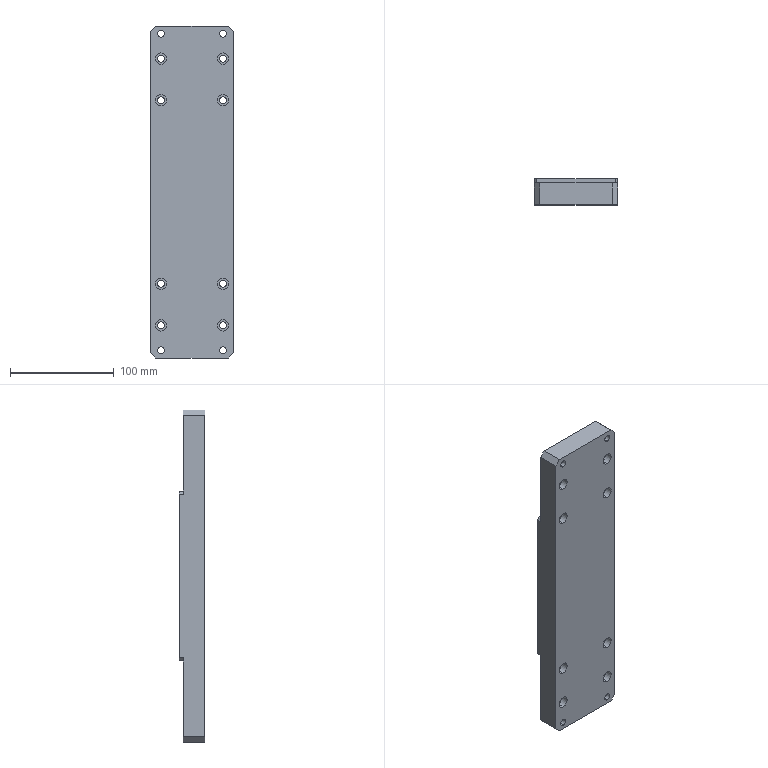CAM job | Mastercam | mm | 14 operations | part box 80 x 25 x 320
1. Contour (2D) | 5 - 10
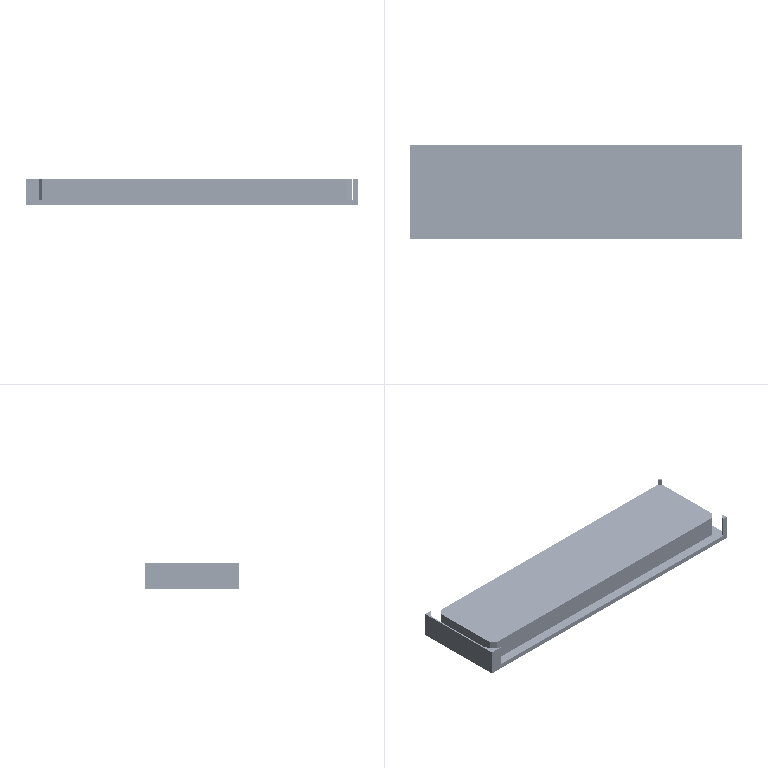2. Surface Rough Pocket | 5 - 10
3. Surface Rough Pocket | 5 - 10
4. Contour (Ramp) | 5 - 10
5. Contour (2D) | 6 - 8
6. Surface Rough Pocket | 6 - 8
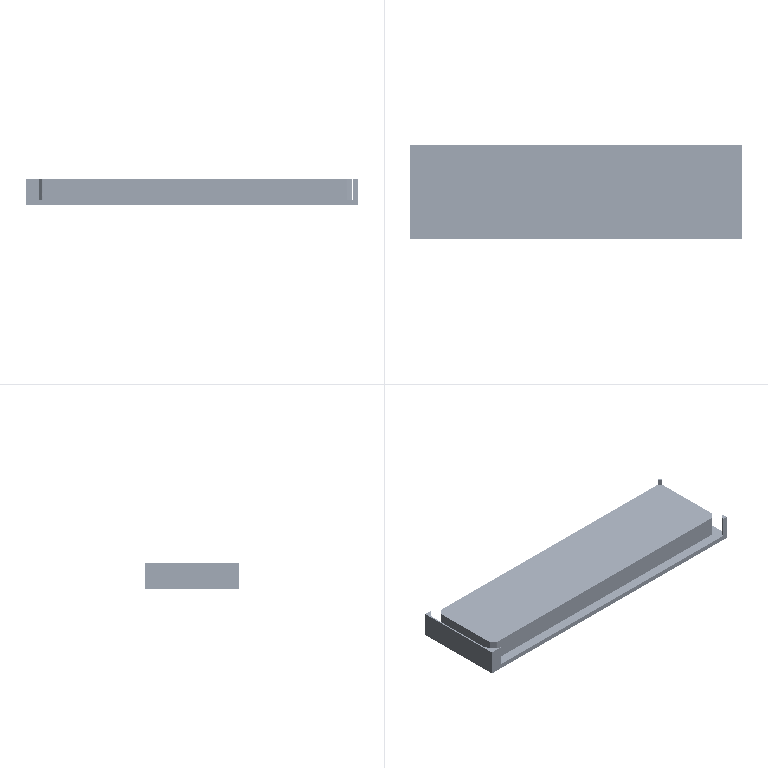7. Facing | 6 - 8
8. Contour (2D) | 6 - 8
9. Contour (Ramp) | 7 - 6
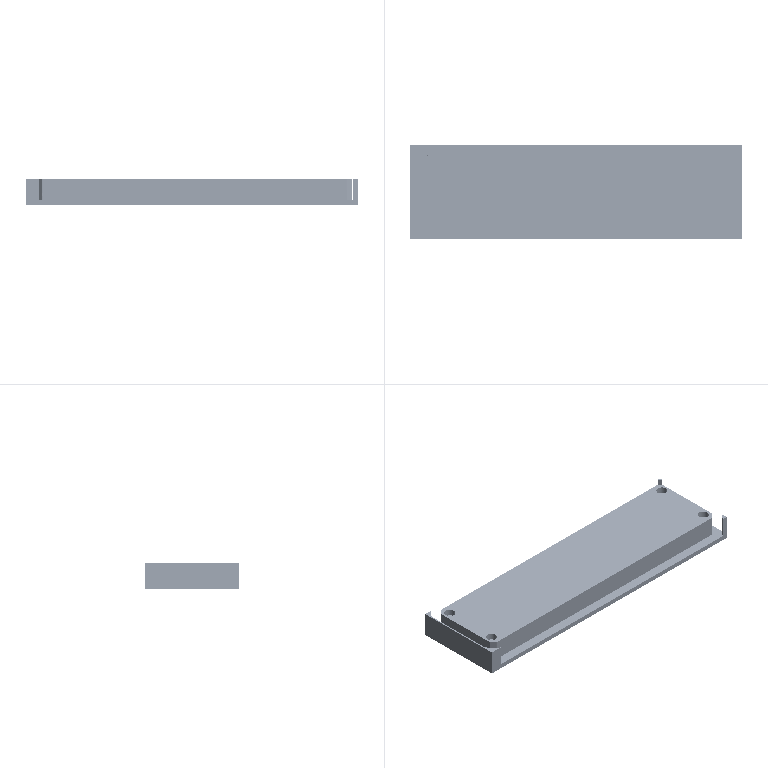10. Drill/Counterbore | 4 - 
11. Drill/Counterbore | 4 - 
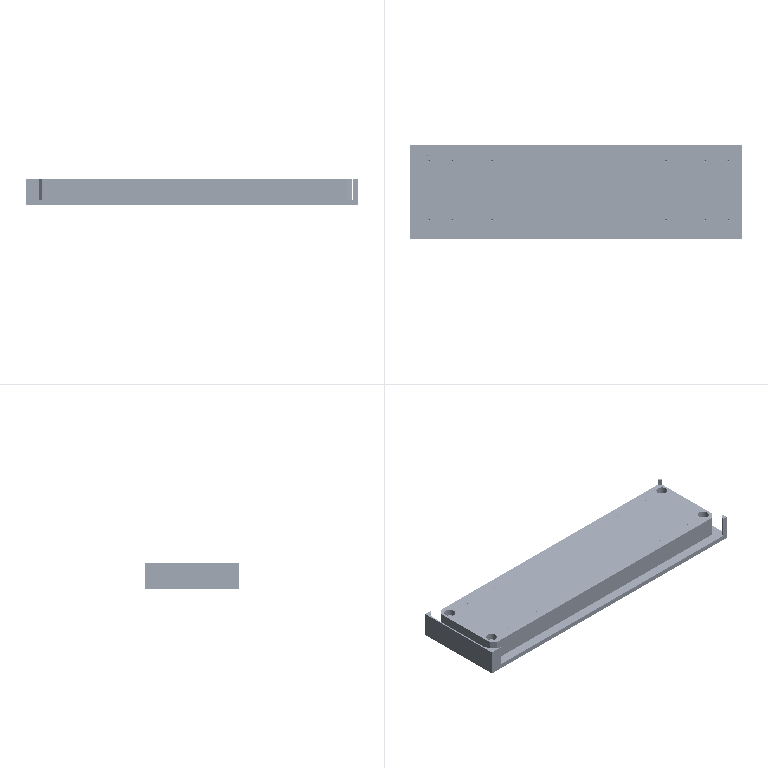12. Contour (2D chamfer) | 4 - 
13. Contour (2D chamfer) | 4 - 
14. Contour (2D chamfer) | 4 - 